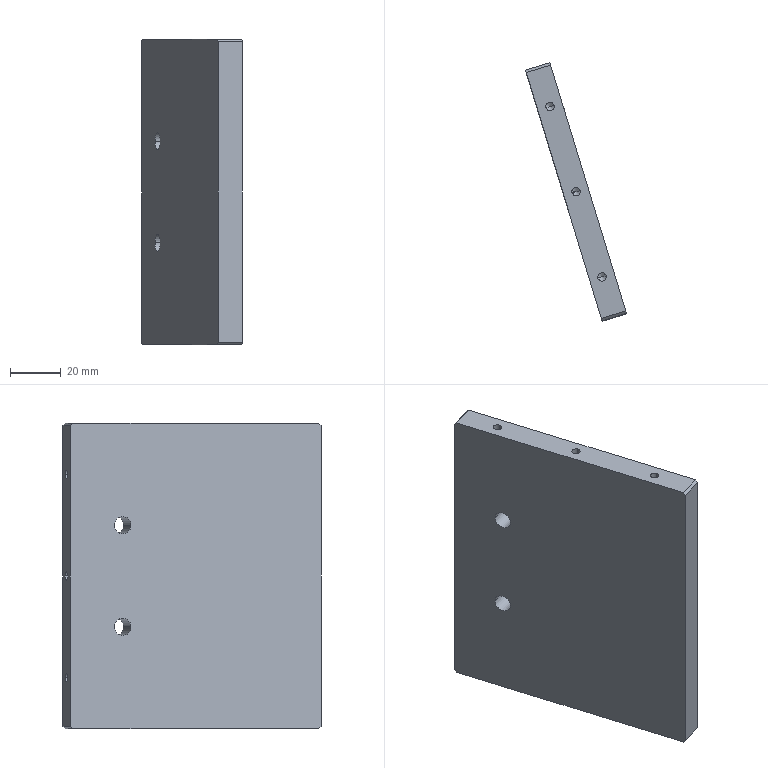Component | SolidWorks | V1ZHXTGrindingBasePlateReinforcementPlateSB1-3 | 1 solid | 38 faces | box 39.62 x 101.43 x 120 mm | volume 122318 mm3 | cylinder 16 | cone 12 | plane 10 | commonest cylinder face diameters 3.3 x12 6.8 x4
build123d program:
from build123d import *

# Parameters (mm, degrees)
SKETCH1_W             = 103
SKETCH1_H             = 120
BOSS_EXTRUDE1_DEPTH   = 5
M4_TAPPED_HOLE1_D     = 3.3
M4_TAPPED_HOLE1_DEPTH = 10.1
M4_TAPPED_HOLE1_TIP   = 0.9914
M4_TAPPED_HOLE2_D     = 3.3
M4_TAPPED_HOLE2_DEPTH = 10.1
M4_TAPPED_HOLE2_TIP   = 0.9914
M8_TAPPED_HOLE1_D     = 6.8
CHAMFER1_SIZE         = 1


with BuildPart() as part:
    # Sketch1 → Boss-Extrude1 (new, symmetric)
    with BuildSketch(Plane.XY):
        Rectangle(SKETCH1_W, SKETCH1_H)
    extrude(amount=BOSS_EXTRUDE1_DEPTH, both=True)

    # M4 Tapped Hole1
    with Locations(Plane.ZY.offset(51.5)):
        with Locations((0, 40), (0, 0), (0, -40)):
            Hole(M4_TAPPED_HOLE1_D / 2, depth=M4_TAPPED_HOLE1_DEPTH)
            with Locations((0, 0, -(M4_TAPPED_HOLE1_DEPTH + M4_TAPPED_HOLE1_TIP / 2))):  # 118° drill point
                Cone(0, M4_TAPPED_HOLE1_D / 2, M4_TAPPED_HOLE1_TIP, mode=Mode.SUBTRACT)

    # M4 Tapped Hole2
    with Locations(Plane(origin=(0, -60, 0), x_dir=(-1, 0, 0), z_dir=(0, -1, 0))):
        with Locations((35, 0), (0, 0), (-35, 0)):
            Hole(M4_TAPPED_HOLE2_D / 2, depth=M4_TAPPED_HOLE2_DEPTH)
            with Locations((0, 0, -(M4_TAPPED_HOLE2_DEPTH + M4_TAPPED_HOLE2_TIP / 2))):  # 118° drill point
                Cone(0, M4_TAPPED_HOLE2_D / 2, M4_TAPPED_HOLE2_TIP, mode=Mode.SUBTRACT)

    # M8 Tapped Hole1 (through all)
    with Locations(Plane(origin=(0, 0, -5), x_dir=(-1, 0, 0), z_dir=(0, 0, -1))):
        with Locations((30, 20), (30, -20)):
            Hole(M8_TAPPED_HOLE1_D / 2)

    # Chamfer1
    chamfer1_edges = [part.edges().sort_by_distance(p)[0] for p in [
        (51.5, -60, 0),
        (-51.5, -60, 0),
        (-51.5, 60, 0),
        (51.5, 60, 0),
    ]]
    chamfer(chamfer1_edges, length=CHAMFER1_SIZE)


solid = part.part

# Placed as in the assembly
solid = solid.moved(Location((115.024, -233.873, 375.239), (-90, 73.032, 0)))
STEP:
#1=COLOUR_RGB('',0.7922,0.8196,0.9333);
#2=FILL_AREA_STYLE_COLOUR('',#1);
#3=FILL_AREA_STYLE('',(#2));
#4=SURFACE_STYLE_FILL_AREA(#3);
#5=SURFACE_SIDE_STYLE('',(#4));
#6=SURFACE_STYLE_USAGE(.BOTH.,#5);
#7=PRESENTATION_STYLE_ASSIGNMENT((#6));
#8=CARTESIAN_POINT('',(4.411,-8.149,13.986));
#9=VERTEX_POINT('',#8);
#10=CARTESIAN_POINT('',(4.333,-7.892,13.986));
#11=VERTEX_POINT('',#10);
#12=CARTESIAN_POINT('',(4.372,-8.02,13.986));
#13=DIRECTION('',(-0.9565,-0.2918,-0.));
#14=DIRECTION('',(-0.2918,0.9565,0.));
#15=AXIS2_PLACEMENT_3D('',#12,#13,#14);
#16=CIRCLE('',#15,0.1339);
#17=EDGE_CURVE('',#9,#11,#16,.T.);
#18=ORIENTED_EDGE('',*,*,#17,.F.);
#19=CARTESIAN_POINT('',(4.035,-8.263,13.986));
#20=VERTEX_POINT('',#19);
#21=CARTESIAN_POINT('',(4.035,-8.263,13.986));
#22=DIRECTION('',(-0.9565,-0.2918,-0.));
#23=VECTOR('',#22,39.37);
#24=LINE('',#21,#23);
#25=EDGE_CURVE('',#9,#20,#24,.T.);
#26=ORIENTED_EDGE('',*,*,#25,.T.);
#27=CARTESIAN_POINT('',(3.956,-8.007,13.986));
#28=VERTEX_POINT('',#27);
#29=CARTESIAN_POINT('',(3.996,-8.135,13.986));
#30=DIRECTION('',(-0.9565,-0.2918,-0.));
#31=DIRECTION('',(-0.2918,0.9565,0.));
#32=AXIS2_PLACEMENT_3D('',#29,#30,#31);
#33=CIRCLE('',#32,0.1339);
#34=EDGE_CURVE('',#20,#28,#33,.T.);
#35=ORIENTED_EDGE('',*,*,#34,.T.);
#36=CARTESIAN_POINT('',(3.956,-8.007,13.986));
#37=DIRECTION('',(-0.9565,-0.2918,-0.));
#38=VECTOR('',#37,39.37);
#39=LINE('',#36,#38);
#40=EDGE_CURVE('',#11,#28,#39,.T.);
#41=ORIENTED_EDGE('',*,*,#40,.F.);
#42=EDGE_LOOP('',(#18,#26,#35,#41));
#43=FACE_OUTER_BOUND('',#42,.T.);
#44=CARTESIAN_POINT('',(3.996,-8.135,13.986));
#45=DIRECTION('',(-0.9565,-0.2918,-0.));
#46=DIRECTION('',(-0.2918,0.9565,0.));
#47=AXIS2_PLACEMENT_3D('',#44,#45,#46);
#48=CYLINDRICAL_SURFACE('',#47,0.1339);
#49=ADVANCED_FACE('',(#43),#48,.F.);
#50=CARTESIAN_POINT('',(4.411,-8.149,15.561));
#51=VERTEX_POINT('',#50);
#52=CARTESIAN_POINT('',(4.333,-7.892,15.561));
#53=VERTEX_POINT('',#52);
#54=CARTESIAN_POINT('',(4.372,-8.02,15.561));
#55=DIRECTION('',(-0.9565,-0.2918,-0.));
#56=DIRECTION('',(-0.2918,0.9565,0.));
#57=AXIS2_PLACEMENT_3D('',#54,#55,#56);
#58=CIRCLE('',#57,0.1339);
#59=EDGE_CURVE('',#51,#53,#58,.T.);
#60=ORIENTED_EDGE('',*,*,#59,.F.);
#61=CARTESIAN_POINT('',(4.035,-8.263,15.561));
#62=VERTEX_POINT('',#61);
#63=CARTESIAN_POINT('',(4.035,-8.263,15.561));
#64=DIRECTION('',(-0.9565,-0.2918,-0.));
#65=VECTOR('',#64,39.37);
#66=LINE('',#63,#65);
#67=EDGE_CURVE('',#51,#62,#66,.T.);
#68=ORIENTED_EDGE('',*,*,#67,.T.);
#69=CARTESIAN_POINT('',(3.956,-8.007,15.561));
#70=VERTEX_POINT('',#69);
#71=CARTESIAN_POINT('',(3.996,-8.135,15.561));
#72=DIRECTION('',(-0.9565,-0.2918,-0.));
#73=DIRECTION('',(-0.2918,0.9565,0.));
#74=AXIS2_PLACEMENT_3D('',#71,#72,#73);
#75=CIRCLE('',#74,0.1339);
#76=EDGE_CURVE('',#62,#70,#75,.T.);
#77=ORIENTED_EDGE('',*,*,#76,.T.);
#78=CARTESIAN_POINT('',(3.956,-8.007,15.561));
#79=DIRECTION('',(-0.9565,-0.2918,-0.));
#80=VECTOR('',#79,39.37);
#81=LINE('',#78,#80);
#82=EDGE_CURVE('',#53,#70,#81,.T.);
#83=ORIENTED_EDGE('',*,*,#82,.F.);
#84=EDGE_LOOP('',(#60,#68,#77,#83));
#85=FACE_OUTER_BOUND('',#84,.T.);
#86=CARTESIAN_POINT('',(3.996,-8.135,15.561));
#87=DIRECTION('',(-0.9565,-0.2918,-0.));
#88=DIRECTION('',(-0.2918,0.9565,0.));
#89=AXIS2_PLACEMENT_3D('',#86,#87,#88);
#90=CYLINDRICAL_SURFACE('',#89,0.1339);
#91=ADVANCED_FACE('',(#85),#90,.F.);
#92=CARTESIAN_POINT('',(4.188,-7.871,16.738));
#93=VERTEX_POINT('',#92);
#94=CARTESIAN_POINT('',(4.064,-7.909,16.738));
#95=VERTEX_POINT('',#94);
#96=CARTESIAN_POINT('',(4.126,-7.89,16.738));
#97=DIRECTION('',(-0.,-0.,1.));
#98=DIRECTION('',(-0.9565,-0.2918,-0.));
#99=AXIS2_PLACEMENT_3D('',#96,#97,#98);
#100=CIRCLE('',#99,0.06496);
#101=EDGE_CURVE('',#93,#95,#100,.T.);
#102=ORIENTED_EDGE('',*,*,#101,.F.);
#103=CARTESIAN_POINT('',(4.188,-7.871,17.135));
#104=VERTEX_POINT('',#103);
#105=CARTESIAN_POINT('',(4.188,-7.871,17.135));
#106=DIRECTION('',(-0.,-0.,1.));
#107=VECTOR('',#106,39.37);
#108=LINE('',#105,#107);
#109=EDGE_CURVE('',#93,#104,#108,.T.);
#110=ORIENTED_EDGE('',*,*,#109,.T.);
#111=CARTESIAN_POINT('',(4.064,-7.909,17.135));
#112=VERTEX_POINT('',#111);
#113=CARTESIAN_POINT('',(4.126,-7.89,17.135));
#114=DIRECTION('',(-0.,-0.,1.));
#115=DIRECTION('',(-0.9565,-0.2918,-0.));
#116=AXIS2_PLACEMENT_3D('',#113,#114,#115);
#117=CIRCLE('',#116,0.06496);
#118=EDGE_CURVE('',#104,#112,#117,.T.);
#119=ORIENTED_EDGE('',*,*,#118,.T.);
#120=CARTESIAN_POINT('',(4.064,-7.909,17.135));
#121=DIRECTION('',(-0.,-0.,1.));
#122=VECTOR('',#121,39.37);
#123=LINE('',#120,#122);
#124=EDGE_CURVE('',#95,#112,#123,.T.);
#125=ORIENTED_EDGE('',*,*,#124,.F.);
#126=EDGE_LOOP('',(#102,#110,#119,#125));
#127=FACE_OUTER_BOUND('',#126,.T.);
#128=CARTESIAN_POINT('',(4.126,-7.89,17.135));
#129=DIRECTION('',(-0.,-0.,1.));
#130=DIRECTION('',(-0.9565,-0.2918,-0.));
#131=AXIS2_PLACEMENT_3D('',#128,#129,#130);
#132=CYLINDRICAL_SURFACE('',#131,0.06496);
#133=ADVANCED_FACE('',(#127),#132,.F.);
#134=CARTESIAN_POINT('',(4.126,-7.89,16.699));
#135=VERTEX_POINT('',#134);
#136=CARTESIAN_POINT('',(4.064,-7.909,16.738));
#137=DIRECTION('',(-0.8199,-0.2501,0.515));
#138=VECTOR('',#137,39.37);
#139=LINE('',#136,#138);
#140=EDGE_CURVE('',#135,#95,#139,.T.);
#141=ORIENTED_EDGE('',*,*,#140,.F.);
#142=CARTESIAN_POINT('',(4.188,-7.871,16.738));
#143=DIRECTION('',(0.8199,0.2501,0.515));
#144=VECTOR('',#143,39.37);
#145=LINE('',#142,#144);
#146=EDGE_CURVE('',#135,#93,#145,.T.);
#147=ORIENTED_EDGE('',*,*,#146,.T.);
#148=ORIENTED_EDGE('',*,*,#101,.T.);
#149=EDGE_LOOP('',(#141,#147,#148));
#150=FACE_OUTER_BOUND('',#149,.T.);
#151=CARTESIAN_POINT('',(4.126,-7.89,16.738));
#152=DIRECTION('',(-0.,-0.,1.));
#153=DIRECTION('',(-0.9565,-0.2918,-0.));
#154=AXIS2_PLACEMENT_3D('',#151,#152,#153);
#155=CONICAL_SURFACE('',#154,0.06496,1.03);
#156=ADVANCED_FACE('',(#150),#155,.F.);
#157=CARTESIAN_POINT('',(4.591,-9.189,16.738));
#158=VERTEX_POINT('',#157);
#159=CARTESIAN_POINT('',(4.466,-9.227,16.738));
#160=VERTEX_POINT('',#159);
#161=CARTESIAN_POINT('',(4.528,-9.208,16.738));
#162=DIRECTION('',(-0.,-0.,1.));
#163=DIRECTION('',(-0.9565,-0.2918,-0.));
#164=AXIS2_PLACEMENT_3D('',#161,#162,#163);
#165=CIRCLE('',#164,0.06496);
#166=EDGE_CURVE('',#158,#160,#165,.T.);
#167=ORIENTED_EDGE('',*,*,#166,.F.);
#168=CARTESIAN_POINT('',(4.591,-9.189,17.135));
#169=VERTEX_POINT('',#168);
#170=CARTESIAN_POINT('',(4.591,-9.189,17.135));
#171=DIRECTION('',(-0.,-0.,1.));
#172=VECTOR('',#171,39.37);
#173=LINE('',#170,#172);
#174=EDGE_CURVE('',#158,#169,#173,.T.);
#175=ORIENTED_EDGE('',*,*,#174,.T.);
#176=CARTESIAN_POINT('',(4.466,-9.227,17.135));
#177=VERTEX_POINT('',#176);
#178=CARTESIAN_POINT('',(4.528,-9.208,17.135));
#179=DIRECTION('',(-0.,-0.,1.));
#180=DIRECTION('',(-0.9565,-0.2918,-0.));
#181=AXIS2_PLACEMENT_3D('',#178,#179,#180);
#182=CIRCLE('',#181,0.06496);
#183=EDGE_CURVE('',#169,#177,#182,.T.);
#184=ORIENTED_EDGE('',*,*,#183,.T.);
#185=CARTESIAN_POINT('',(4.466,-9.227,17.135));
#186=DIRECTION('',(-0.,-0.,1.));
#187=VECTOR('',#186,39.37);
#188=LINE('',#185,#187);
#189=EDGE_CURVE('',#160,#177,#188,.T.);
#190=ORIENTED_EDGE('',*,*,#189,.F.);
#191=EDGE_LOOP('',(#167,#175,#184,#190));
#192=FACE_OUTER_BOUND('',#191,.T.);
#193=CARTESIAN_POINT('',(4.528,-9.208,17.135));
#194=DIRECTION('',(-0.,-0.,1.));
#195=DIRECTION('',(-0.9565,-0.2918,-0.));
#196=AXIS2_PLACEMENT_3D('',#193,#194,#195);
#197=CYLINDRICAL_SURFACE('',#196,0.06496);
#198=ADVANCED_FACE('',(#192),#197,.F.);
#199=CARTESIAN_POINT('',(4.528,-9.208,16.699));
#200=VERTEX_POINT('',#199);
#201=CARTESIAN_POINT('',(4.466,-9.227,16.738));
#202=DIRECTION('',(-0.8199,-0.2501,0.515));
#203=VECTOR('',#202,39.37);
#204=LINE('',#201,#203);
#205=EDGE_CURVE('',#200,#160,#204,.T.);
#206=ORIENTED_EDGE('',*,*,#205,.F.);
#207=CARTESIAN_POINT('',(4.591,-9.189,16.738));
#208=DIRECTION('',(0.8199,0.2501,0.515));
#209=VECTOR('',#208,39.37);
#210=LINE('',#207,#209);
#211=EDGE_CURVE('',#200,#158,#210,.T.);
#212=ORIENTED_EDGE('',*,*,#211,.T.);
#213=ORIENTED_EDGE('',*,*,#166,.T.);
#214=EDGE_LOOP('',(#206,#212,#213));
#215=FACE_OUTER_BOUND('',#214,.T.);
#216=CARTESIAN_POINT('',(4.528,-9.208,16.738));
#217=DIRECTION('',(-0.,-0.,1.));
#218=DIRECTION('',(-0.9565,-0.2918,-0.));
#219=AXIS2_PLACEMENT_3D('',#216,#217,#218);
#220=CONICAL_SURFACE('',#219,0.06496,1.03);
#221=ADVANCED_FACE('',(#215),#220,.F.);
#222=CARTESIAN_POINT('',(4.993,-10.507,16.738));
#223=VERTEX_POINT('',#222);
#224=CARTESIAN_POINT('',(4.868,-10.545,16.738));
#225=VERTEX_POINT('',#224);
#226=CARTESIAN_POINT('',(4.931,-10.526,16.738));
#227=DIRECTION('',(-0.,-0.,1.));
#228=DIRECTION('',(-0.9565,-0.2918,-0.));
#229=AXIS2_PLACEMENT_3D('',#226,#227,#228);
#230=CIRCLE('',#229,0.06496);
#231=EDGE_CURVE('',#223,#225,#230,.T.);
#232=ORIENTED_EDGE('',*,*,#231,.F.);
#233=CARTESIAN_POINT('',(4.993,-10.507,17.135));
#234=VERTEX_POINT('',#233);
#235=CARTESIAN_POINT('',(4.993,-10.507,17.135));
#236=DIRECTION('',(-0.,-0.,1.));
#237=VECTOR('',#236,39.37);
#238=LINE('',#235,#237);
#239=EDGE_CURVE('',#223,#234,#238,.T.);
#240=ORIENTED_EDGE('',*,*,#239,.T.);
#241=CARTESIAN_POINT('',(4.868,-10.545,17.135));
#242=VERTEX_POINT('',#241);
#243=CARTESIAN_POINT('',(4.931,-10.526,17.135));
#244=DIRECTION('',(-0.,-0.,1.));
#245=DIRECTION('',(-0.9565,-0.2918,-0.));
#246=AXIS2_PLACEMENT_3D('',#243,#244,#245);
#247=CIRCLE('',#246,0.06496);
#248=EDGE_CURVE('',#234,#242,#247,.T.);
#249=ORIENTED_EDGE('',*,*,#248,.T.);
#250=CARTESIAN_POINT('',(4.868,-10.545,17.135));
#251=DIRECTION('',(-0.,-0.,1.));
#252=VECTOR('',#251,39.37);
#253=LINE('',#250,#252);
#254=EDGE_CURVE('',#225,#242,#253,.T.);
#255=ORIENTED_EDGE('',*,*,#254,.F.);
#256=EDGE_LOOP('',(#232,#240,#249,#255));
#257=FACE_OUTER_BOUND('',#256,.T.);
#258=CARTESIAN_POINT('',(4.931,-10.526,17.135));
#259=DIRECTION('',(-0.,-0.,1.));
#260=DIRECTION('',(-0.9565,-0.2918,-0.));
#261=AXIS2_PLACEMENT_3D('',#258,#259,#260);
#262=CYLINDRICAL_SURFACE('',#261,0.06496);
#263=ADVANCED_FACE('',(#257),#262,.F.);
#264=CARTESIAN_POINT('',(4.931,-10.526,16.699));
#265=VERTEX_POINT('',#264);
#266=CARTESIAN_POINT('',(4.868,-10.545,16.738));
#267=DIRECTION('',(-0.8199,-0.2501,0.515));
#268=VECTOR('',#267,39.37);
#269=LINE('',#266,#268);
#270=EDGE_CURVE('',#265,#225,#269,.T.);
#271=ORIENTED_EDGE('',*,*,#270,.F.);
#272=CARTESIAN_POINT('',(4.993,-10.507,16.738));
#273=DIRECTION('',(0.8199,0.2501,0.515));
#274=VECTOR('',#273,39.37);
#275=LINE('',#272,#274);
#276=EDGE_CURVE('',#265,#223,#275,.T.);
#277=ORIENTED_EDGE('',*,*,#276,.T.);
#278=ORIENTED_EDGE('',*,*,#231,.T.);
#279=EDGE_LOOP('',(#271,#277,#278));
#280=FACE_OUTER_BOUND('',#279,.T.);
#281=CARTESIAN_POINT('',(4.931,-10.526,16.738));
#282=DIRECTION('',(-0.,-0.,1.));
#283=DIRECTION('',(-0.9565,-0.2918,-0.));
#284=AXIS2_PLACEMENT_3D('',#281,#282,#283);
#285=CONICAL_SURFACE('',#284,0.06496,1.03);
#286=ADVANCED_FACE('',(#280),#285,.F.);
#287=CARTESIAN_POINT('',(3.991,-7.668,13.198));
#288=VERTEX_POINT('',#287);
#289=CARTESIAN_POINT('',(4.115,-7.63,13.198));
#290=VERTEX_POINT('',#289);
#291=CARTESIAN_POINT('',(4.053,-7.649,13.198));
#292=DIRECTION('',(-0.2918,0.9565,0.));
#293=DIRECTION('',(0.9565,0.2918,0.));
#294=AXIS2_PLACEMENT_3D('',#291,#292,#293);
#295=CIRCLE('',#294,0.06496);
#296=EDGE_CURVE('',#288,#290,#295,.T.);
#297=ORIENTED_EDGE('',*,*,#296,.F.);
#298=CARTESIAN_POINT('',(3.875,-7.287,13.198));
#299=VERTEX_POINT('',#298);
#300=CARTESIAN_POINT('',(3.875,-7.287,13.198));
#301=DIRECTION('',(-0.2918,0.9565,0.));
#302=VECTOR('',#301,39.37);
#303=LINE('',#300,#302);
#304=EDGE_CURVE('',#288,#299,#303,.T.);
#305=ORIENTED_EDGE('',*,*,#304,.T.);
#306=CARTESIAN_POINT('',(3.999,-7.249,13.198));
#307=VERTEX_POINT('',#306);
#308=CARTESIAN_POINT('',(3.937,-7.268,13.198));
#309=DIRECTION('',(-0.2918,0.9565,0.));
#310=DIRECTION('',(0.9565,0.2918,0.));
#311=AXIS2_PLACEMENT_3D('',#308,#309,#310);
#312=CIRCLE('',#311,0.06496);
#313=EDGE_CURVE('',#299,#307,#312,.T.);
#314=ORIENTED_EDGE('',*,*,#313,.T.);
#315=CARTESIAN_POINT('',(3.999,-7.249,13.198));
#316=DIRECTION('',(-0.2918,0.9565,0.));
#317=VECTOR('',#316,39.37);
#318=LINE('',#315,#317);
#319=EDGE_CURVE('',#290,#307,#318,.T.);
#320=ORIENTED_EDGE('',*,*,#319,.F.);
#321=EDGE_LOOP('',(#297,#305,#314,#320));
#322=FACE_OUTER_BOUND('',#321,.T.);
#323=CARTESIAN_POINT('',(3.937,-7.268,13.198));
#324=DIRECTION('',(-0.2918,0.9565,0.));
#325=DIRECTION('',(0.9565,0.2918,0.));
#326=AXIS2_PLACEMENT_3D('',#323,#324,#325);
#327=CYLINDRICAL_SURFACE('',#326,0.06496);
#328=ADVANCED_FACE('',(#322),#327,.F.);
#329=CARTESIAN_POINT('',(4.064,-7.686,13.198));
#330=VERTEX_POINT('',#329);
#331=CARTESIAN_POINT('',(4.115,-7.63,13.198));
#332=DIRECTION('',(0.6696,0.7428,0.));
#333=VECTOR('',#332,39.37);
#334=LINE('',#331,#333);
#335=EDGE_CURVE('',#330,#290,#334,.T.);
#336=ORIENTED_EDGE('',*,*,#335,.F.);
#337=CARTESIAN_POINT('',(3.991,-7.668,13.198));
#338=DIRECTION('',(-0.9702,0.2425,0.));
#339=VECTOR('',#338,39.37);
#340=LINE('',#337,#339);
#341=EDGE_CURVE('',#330,#288,#340,.T.);
#342=ORIENTED_EDGE('',*,*,#341,.T.);
#343=ORIENTED_EDGE('',*,*,#296,.T.);
#344=EDGE_LOOP('',(#336,#342,#343));
#345=FACE_OUTER_BOUND('',#344,.T.);
#346=CARTESIAN_POINT('',(4.053,-7.649,13.198));
#347=DIRECTION('',(-0.2918,0.9565,0.));
#348=DIRECTION('',(0.9565,0.2918,0.));
#349=AXIS2_PLACEMENT_3D('',#346,#347,#348);
#350=CONICAL_SURFACE('',#349,0.06496,1.03);
#351=ADVANCED_FACE('',(#345),#350,.F.);
#352=CARTESIAN_POINT('',(3.991,-7.668,14.773));
#353=VERTEX_POINT('',#352);
#354=CARTESIAN_POINT('',(4.115,-7.63,14.773));
#355=VERTEX_POINT('',#354);
#356=CARTESIAN_POINT('',(4.053,-7.649,14.773));
#357=DIRECTION('',(-0.2918,0.9565,0.));
#358=DIRECTION('',(0.9565,0.2918,0.));
#359=AXIS2_PLACEMENT_3D('',#356,#357,#358);
#360=CIRCLE('',#359,0.06496);
#361=EDGE_CURVE('',#353,#355,#360,.T.);
#362=ORIENTED_EDGE('',*,*,#361,.F.);
#363=CARTESIAN_POINT('',(3.875,-7.287,14.773));
#364=VERTEX_POINT('',#363);
#365=CARTESIAN_POINT('',(3.875,-7.287,14.773));
#366=DIRECTION('',(-0.2918,0.9565,0.));
#367=VECTOR('',#366,39.37);
#368=LINE('',#365,#367);
#369=EDGE_CURVE('',#353,#364,#368,.T.);
#370=ORIENTED_EDGE('',*,*,#369,.T.);
#371=CARTESIAN_POINT('',(3.999,-7.249,14.773));
#372=VERTEX_POINT('',#371);
#373=CARTESIAN_POINT('',(3.937,-7.268,14.773));
#374=DIRECTION('',(-0.2918,0.9565,0.));
#375=DIRECTION('',(0.9565,0.2918,0.));
#376=AXIS2_PLACEMENT_3D('',#373,#374,#375);
#377=CIRCLE('',#376,0.06496);
#378=EDGE_CURVE('',#364,#372,#377,.T.);
#379=ORIENTED_EDGE('',*,*,#378,.T.);
#380=CARTESIAN_POINT('',(3.999,-7.249,14.773));
#381=DIRECTION('',(-0.2918,0.9565,0.));
#382=VECTOR('',#381,39.37);
#383=LINE('',#380,#382);
#384=EDGE_CURVE('',#355,#372,#383,.T.);
#385=ORIENTED_EDGE('',*,*,#384,.F.);
#386=EDGE_LOOP('',(#362,#370,#379,#385));
#387=FACE_OUTER_BOUND('',#386,.T.);
#388=CARTESIAN_POINT('',(3.937,-7.268,14.773));
#389=DIRECTION('',(-0.2918,0.9565,0.));
#390=DIRECTION('',(0.9565,0.2918,0.));
#391=AXIS2_PLACEMENT_3D('',#388,#389,#390);
#392=CYLINDRICAL_SURFACE('',#391,0.06496);
#393=ADVANCED_FACE('',(#387),#392,.F.);
#394=CARTESIAN_POINT('',(4.064,-7.686,14.773));
#395=VERTEX_POINT('',#394);
#396=CARTESIAN_POINT('',(4.115,-7.63,14.773));
#397=DIRECTION('',(0.6696,0.7428,0.));
#398=VECTOR('',#397,39.37);
#399=LINE('',#396,#398);
#400=EDGE_CURVE('',#395,#355,#399,.T.);
#401=ORIENTED_EDGE('',*,*,#400,.F.);
#402=CARTESIAN_POINT('',(3.991,-7.668,14.773));
#403=DIRECTION('',(-0.9702,0.2425,0.));
#404=VECTOR('',#403,39.37);
#405=LINE('',#402,#404);
#406=EDGE_CURVE('',#395,#353,#405,.T.);
#407=ORIENTED_EDGE('',*,*,#406,.T.);
#408=ORIENTED_EDGE('',*,*,#361,.T.);
#409=EDGE_LOOP('',(#401,#407,#408));
#410=FACE_OUTER_BOUND('',#409,.T.);
#411=CARTESIAN_POINT('',(4.053,-7.649,14.773));
#412=DIRECTION('',(-0.2918,0.9565,0.));
#413=DIRECTION('',(0.9565,0.2918,0.));
#414=AXIS2_PLACEMENT_3D('',#411,#412,#413);
#415=CONICAL_SURFACE('',#414,0.06496,1.03);
#416=ADVANCED_FACE('',(#410),#415,.F.);
#417=CARTESIAN_POINT('',(3.991,-7.668,16.348));
#418=VERTEX_POINT('',#417);
#419=CARTESIAN_POINT('',(4.115,-7.63,16.348));
#420=VERTEX_POINT('',#419);
#421=CARTESIAN_POINT('',(4.053,-7.649,16.348));
#422=DIRECTION('',(-0.2918,0.9565,0.));
#423=DIRECTION('',(0.9565,0.2918,0.));
#424=AXIS2_PLACEMENT_3D('',#421,#422,#423);
#425=CIRCLE('',#424,0.06496);
#426=EDGE_CURVE('',#418,#420,#425,.T.);
#427=ORIENTED_EDGE('',*,*,#426,.F.);
#428=CARTESIAN_POINT('',(3.875,-7.287,16.348));
#429=VERTEX_POINT('',#428);
#430=CARTESIAN_POINT('',(3.875,-7.287,16.348));
#431=DIRECTION('',(-0.2918,0.9565,0.));
#432=VECTOR('',#431,39.37);
#433=LINE('',#430,#432);
#434=EDGE_CURVE('',#418,#429,#433,.T.);
#435=ORIENTED_EDGE('',*,*,#434,.T.);
#436=CARTESIAN_POINT('',(3.999,-7.249,16.348));
#437=VERTEX_POINT('',#436);
#438=CARTESIAN_POINT('',(3.937,-7.268,16.348));
#439=DIRECTION('',(-0.2918,0.9565,0.));
#440=DIRECTION('',(0.9565,0.2918,0.));
#441=AXIS2_PLACEMENT_3D('',#438,#439,#440);
#442=CIRCLE('',#441,0.06496);
#443=EDGE_CURVE('',#429,#437,#442,.T.);
#444=ORIENTED_EDGE('',*,*,#443,.T.);
#445=CARTESIAN_POINT('',(3.999,-7.249,16.348));
#446=DIRECTION('',(-0.2918,0.9565,0.));
#447=VECTOR('',#446,39.37);
#448=LINE('',#445,#447);
#449=EDGE_CURVE('',#420,#437,#448,.T.);
#450=ORIENTED_EDGE('',*,*,#449,.F.);
#451=EDGE_LOOP('',(#427,#435,#444,#450));
#452=FACE_OUTER_BOUND('',#451,.T.);
#453=CARTESIAN_POINT('',(3.937,-7.268,16.348));
#454=DIRECTION('',(-0.2918,0.9565,0.));
#455=DIRECTION('',(0.9565,0.2918,0.));
#456=AXIS2_PLACEMENT_3D('',#453,#454,#455);
#457=CYLINDRICAL_SURFACE('',#456,0.06496);
#458=ADVANCED_FACE('',(#452),#457,.F.);
#459=CARTESIAN_POINT('',(4.064,-7.686,16.348));
#460=VERTEX_POINT('',#459);
#461=CARTESIAN_POINT('',(4.115,-7.63,16.348));
#462=DIRECTION('',(0.6696,0.7428,0.));
#463=VECTOR('',#462,39.37);
#464=LINE('',#461,#463);
#465=EDGE_CURVE('',#460,#420,#464,.T.);
#466=ORIENTED_EDGE('',*,*,#465,.F.);
#467=CARTESIAN_POINT('',(3.991,-7.668,16.348));
#468=DIRECTION('',(-0.9702,0.2425,0.));
#469=VECTOR('',#468,39.37);
#470=LINE('',#467,#469);
#471=EDGE_CURVE('',#460,#418,#470,.T.);
#472=ORIENTED_EDGE('',*,*,#471,.T.);
#473=ORIENTED_EDGE('',*,*,#426,.T.);
#474=EDGE_LOOP('',(#466,#472,#473));
#475=FACE_OUTER_BOUND('',#474,.T.);
#476=CARTESIAN_POINT('',(4.053,-7.649,16.348));
#477=DIRECTION('',(-0.2918,0.9565,0.));
#478=DIRECTION('',(0.9565,0.2918,0.));
#479=AXIS2_PLACEMENT_3D('',#476,#477,#478);
#480=CONICAL_SURFACE('',#479,0.06496,1.03);
#481=ADVANCED_FACE('',(#475),#480,.F.);
#482=CARTESIAN_POINT('',(5.308,-11.089,17.096));
#483=VERTEX_POINT('',#482);
#484=CARTESIAN_POINT('',(5.308,-11.089,12.45));
#485=VERTEX_POINT('',#484);
#486=CARTESIAN_POINT('',(5.308,-11.089,17.135));
#487=DIRECTION('',(0.,0.,-1.));
#488=VECTOR('',#487,39.37);
#489=LINE('',#486,#488);
#490=EDGE_CURVE('',#483,#485,#489,.T.);
#491=ORIENTED_EDGE('',*,*,#490,.F.);
#492=CARTESIAN_POINT('',(4.932,-11.204,17.096));
#493=VERTEX_POINT('',#492);
#494=CARTESIAN_POINT('',(5.308,-11.089,17.096));
#495=DIRECTION('',(-0.9565,-0.2918,-0.));
#496=VECTOR('',#495,39.37);
#497=LINE('',#494,#496);
#498=EDGE_CURVE('',#483,#493,#497,.T.);
#499=ORIENTED_EDGE('',*,*,#498,.T.);
#500=CARTESIAN_POINT('',(4.932,-11.204,12.45));
#501=VERTEX_POINT('',#500);
#502=CARTESIAN_POINT('',(4.932,-11.204,17.135));
#503=DIRECTION('',(0.,0.,-1.));
#504=VECTOR('',#503,39.37);
#505=LINE('',#502,#504);
#506=EDGE_CURVE('',#493,#501,#505,.T.);
#507=ORIENTED_EDGE('',*,*,#506,.T.);
#508=CARTESIAN_POINT('',(5.308,-11.089,12.45));
#509=DIRECTION('',(0.9565,0.2918,0.));
#510=VECTOR('',#509,39.37);
#511=LINE('',#508,#510);
#512=EDGE_CURVE('',#501,#485,#511,.T.);
#513=ORIENTED_EDGE('',*,*,#512,.T.);
#514=EDGE_LOOP('',(#491,#499,#507,#513));
#515=FACE_OUTER_BOUND('',#514,.T.);
#516=CARTESIAN_POINT('',(5.308,-11.089,17.135));
#517=DIRECTION('',(-0.2918,0.9565,0.));
#518=DIRECTION('',(0.9565,0.2918,0.));
#519=AXIS2_PLACEMENT_3D('',#516,#517,#518);
#520=PLANE('',#519);
#521=ADVANCED_FACE('',(#515),#520,.F.);
#522=CARTESIAN_POINT('',(5.297,-11.052,12.411));
#523=VERTEX_POINT('',#522);
#524=CARTESIAN_POINT('',(4.137,-7.249,12.411));
#525=VERTEX_POINT('',#524);
#526=CARTESIAN_POINT('',(4.125,-7.211,12.411));
#527=DIRECTION('',(-0.2918,0.9565,0.));
#528=VECTOR('',#527,39.37);
#529=LINE('',#526,#528);
#530=EDGE_CURVE('',#523,#525,#529,.T.);
#531=ORIENTED_EDGE('',*,*,#530,.F.);
#532=CARTESIAN_POINT('',(4.92,-11.167,12.411));
#533=VERTEX_POINT('',#532);
#534=CARTESIAN_POINT('',(5.297,-11.052,12.411));
#535=DIRECTION('',(-0.9565,-0.2918,-0.));
#536=VECTOR('',#535,39.37);
#537=LINE('',#534,#536);
#538=EDGE_CURVE('',#523,#533,#537,.T.);
#539=ORIENTED_EDGE('',*,*,#538,.T.);
#540=CARTESIAN_POINT('',(3.76,-7.363,12.411));
#541=VERTEX_POINT('',#540);
#542=CARTESIAN_POINT('',(3.749,-7.326,12.411));
#543=DIRECTION('',(-0.2918,0.9565,0.));
#544=VECTOR('',#543,39.37);
#545=LINE('',#542,#544);
#546=EDGE_CURVE('',#533,#541,#545,.T.);
#547=ORIENTED_EDGE('',*,*,#546,.T.);
#548=CARTESIAN_POINT('',(4.137,-7.249,12.411));
#549=DIRECTION('',(0.9565,0.2918,0.));
#550=VECTOR('',#549,39.37);
#551=LINE('',#548,#550);
#552=EDGE_CURVE('',#541,#525,#551,.T.);
#553=ORIENTED_EDGE('',*,*,#552,.T.);
#554=EDGE_LOOP('',(#531,#539,#547,#553));
#555=FACE_OUTER_BOUND('',#554,.T.);
#556=CARTESIAN_POINT('',(4.125,-7.211,12.411));
#557=DIRECTION('',(-0.,-0.,1.));
#558=DIRECTION('',(-0.9565,-0.2918,-0.));
#559=AXIS2_PLACEMENT_3D('',#556,#557,#558);
#560=PLANE('',#559);
#561=ADVANCED_FACE('',(#555),#560,.F.);
#562=CARTESIAN_POINT('',(3.937,-7.268,13.198));
#563=DIRECTION('',(-0.2918,0.9565,0.));
#564=DIRECTION('',(0.9565,0.2918,0.));
#565=AXIS2_PLACEMENT_3D('',#562,#563,#564);
#566=CIRCLE('',#565,0.06496);
#567=EDGE_CURVE('',#307,#299,#566,.T.);
#568=ORIENTED_EDGE('',*,*,#567,.F.);
#569=ORIENTED_EDGE('',*,*,#313,.F.);
#570=EDGE_LOOP('',(#568,#569));
#571=FACE_BOUND('',#570,.T.);
#572=CARTESIAN_POINT('',(3.937,-7.268,14.773));
#573=DIRECTION('',(-0.2918,0.9565,0.));
#574=DIRECTION('',(0.9565,0.2918,0.));
#575=AXIS2_PLACEMENT_3D('',#572,#573,#574);
#576=CIRCLE('',#575,0.06496);
#577=EDGE_CURVE('',#372,#364,#576,.T.);
#578=ORIENTED_EDGE('',*,*,#577,.F.);
#579=ORIENTED_EDGE('',*,*,#378,.F.);
#580=EDGE_LOOP('',(#578,#579));
#581=FACE_BOUND('',#580,.T.);
#582=CARTESIAN_POINT('',(3.937,-7.268,16.348));
#583=DIRECTION('',(-0.2918,0.9565,0.));
#584=DIRECTION('',(0.9565,0.2918,0.));
#585=AXIS2_PLACEMENT_3D('',#582,#583,#584);
#586=CIRCLE('',#585,0.06496);
#587=EDGE_CURVE('',#437,#429,#586,.T.);
#588=ORIENTED_EDGE('',*,*,#587,.F.);
#589=ORIENTED_EDGE('',*,*,#443,.F.);
#590=EDGE_LOOP('',(#588,#589));
#591=FACE_BOUND('',#590,.T.);
#592=CARTESIAN_POINT('',(3.749,-7.326,12.45));
#593=VERTEX_POINT('',#592);
#594=CARTESIAN_POINT('',(3.749,-7.326,17.096));
#595=VERTEX_POINT('',#594);
#596=CARTESIAN_POINT('',(3.749,-7.326,17.135));
#597=DIRECTION('',(-0.,-0.,1.));
#598=VECTOR('',#597,39.37);
#599=LINE('',#596,#598);
#600=EDGE_CURVE('',#593,#595,#599,.T.);
#601=ORIENTED_EDGE('',*,*,#600,.T.);
#602=CARTESIAN_POINT('',(4.125,-7.211,17.096));
#603=VERTEX_POINT('',#602);
#604=CARTESIAN_POINT('',(4.125,-7.211,17.096));
#605=DIRECTION('',(0.9565,0.2918,0.));
#606=VECTOR('',#605,39.37);
#607=LINE('',#604,#606);
#608=EDGE_CURVE('',#595,#603,#607,.T.);
#609=ORIENTED_EDGE('',*,*,#608,.T.);
#610=CARTESIAN_POINT('',(4.125,-7.211,12.45));
#611=VERTEX_POINT('',#610);
#612=CARTESIAN_POINT('',(4.125,-7.211,17.135));
#613=DIRECTION('',(-0.,-0.,1.));
#614=VECTOR('',#613,39.37);
#615=LINE('',#612,#614);
#616=EDGE_CURVE('',#611,#603,#615,.T.);
#617=ORIENTED_EDGE('',*,*,#616,.F.);
#618=CARTESIAN_POINT('',(4.125,-7.211,12.45));
#619=DIRECTION('',(-0.9565,-0.2918,-0.));
#620=VECTOR('',#619,39.37);
#621=LINE('',#618,#620);
#622=EDGE_CURVE('',#611,#593,#621,.T.);
#623=ORIENTED_EDGE('',*,*,#622,.T.);
#624=EDGE_LOOP('',(#601,#609,#617,#623));
#625=FACE_OUTER_BOUND('',#624,.T.);
#626=CARTESIAN_POINT('',(4.125,-7.211,17.135));
#627=DIRECTION('',(0.2918,-0.9565,-0.));
#628=DIRECTION('',(-0.9565,-0.2918,-0.));
#629=AXIS2_PLACEMENT_3D('',#626,#627,#628);
#630=PLANE('',#629);
#631=ADVANCED_FACE('',(#571,#581,#591,#625),#630,.F.);
#632=CARTESIAN_POINT('',(4.126,-7.89,17.135));
#633=DIRECTION('',(-0.,-0.,1.));
#634=DIRECTION('',(-0.9565,-0.2918,-0.));
#635=AXIS2_PLACEMENT_3D('',#632,#633,#634);
#636=CIRCLE('',#635,0.06496);
#637=EDGE_CURVE('',#112,#104,#636,.T.);
#638=ORIENTED_EDGE('',*,*,#637,.F.);
#639=ORIENTED_EDGE('',*,*,#118,.F.);
#640=EDGE_LOOP('',(#638,#639));
#641=FACE_BOUND('',#640,.T.);
#642=CARTESIAN_POINT('',(4.528,-9.208,17.135));
#643=DIRECTION('',(-0.,-0.,1.));
#644=DIRECTION('',(-0.9565,-0.2918,-0.));
#645=AXIS2_PLACEMENT_3D('',#642,#643,#644);
#646=CIRCLE('',#645,0.06496);
#647=EDGE_CURVE('',#177,#169,#646,.T.);
#648=ORIENTED_EDGE('',*,*,#647,.F.);
#649=ORIENTED_EDGE('',*,*,#183,.F.);
#650=EDGE_LOOP('',(#648,#649));
#651=FACE_BOUND('',#650,.T.);
#652=CARTESIAN_POINT('',(4.931,-10.526,17.135));
#653=DIRECTION('',(-0.,-0.,1.));
#654=DIRECTION('',(-0.9565,-0.2918,-0.));
#655=AXIS2_PLACEMENT_3D('',#652,#653,#654);
#656=CIRCLE('',#655,0.06496);
#657=EDGE_CURVE('',#242,#234,#656,.T.);
#658=ORIENTED_EDGE('',*,*,#657,.F.);
#659=ORIENTED_EDGE('',*,*,#248,.F.);
#660=EDGE_LOOP('',(#658,#659));
#661=FACE_BOUND('',#660,.T.);
#662=CARTESIAN_POINT('',(4.137,-7.249,17.135));
#663=VERTEX_POINT('',#662);
#664=CARTESIAN_POINT('',(5.297,-11.052,17.135));
#665=VERTEX_POINT('',#664);
#666=CARTESIAN_POINT('',(4.125,-7.211,17.135));
#667=DIRECTION('',(0.2918,-0.9565,-0.));
#668=VECTOR('',#667,39.37);
#669=LINE('',#666,#668);
#670=EDGE_CURVE('',#663,#665,#669,.T.);
#671=ORIENTED_EDGE('',*,*,#670,.F.);
#672=CARTESIAN_POINT('',(3.76,-7.363,17.135));
#673=VERTEX_POINT('',#672);
#674=CARTESIAN_POINT('',(4.137,-7.249,17.135));
#675=DIRECTION('',(-0.9565,-0.2918,-0.));
#676=VECTOR('',#675,39.37);
#677=LINE('',#674,#676);
#678=EDGE_CURVE('',#663,#673,#677,.T.);
#679=ORIENTED_EDGE('',*,*,#678,.T.);
#680=CARTESIAN_POINT('',(4.92,-11.167,17.135));
#681=VERTEX_POINT('',#680);
#682=CARTESIAN_POINT('',(3.749,-7.326,17.135));
#683=DIRECTION('',(0.2918,-0.9565,-0.));
#684=VECTOR('',#683,39.37);
#685=LINE('',#682,#684);
#686=EDGE_CURVE('',#673,#681,#685,.T.);
#687=ORIENTED_EDGE('',*,*,#686,.T.);
#688=CARTESIAN_POINT('',(5.297,-11.052,17.135));
#689=DIRECTION('',(0.9565,0.2918,0.));
#690=VECTOR('',#689,39.37);
#691=LINE('',#688,#690);
#692=EDGE_CURVE('',#681,#665,#691,.T.);
#693=ORIENTED_EDGE('',*,*,#692,.T.);
#694=EDGE_LOOP('',(#671,#679,#687,#693));
#695=FACE_OUTER_BOUND('',#694,.T.);
#696=CARTESIAN_POINT('',(4.125,-7.211,17.135));
#697=DIRECTION('',(0.,0.,-1.));
#698=DIRECTION('',(0.9565,0.2918,0.));
#699=AXIS2_PLACEMENT_3D('',#696,#697,#698);
#700=PLANE('',#699);
#701=ADVANCED_FACE('',(#641,#651,#661,#695),#700,.F.);
#702=CARTESIAN_POINT('',(4.372,-8.02,13.986));
#703=DIRECTION('',(-0.9565,-0.2918,-0.));
#704=DIRECTION('',(-0.2918,0.9565,0.));
#705=AXIS2_PLACEMENT_3D('',#702,#703,#704);
#706=CIRCLE('',#705,0.1339);
#707=EDGE_CURVE('',#11,#9,#706,.T.);
#708=ORIENTED_EDGE('',*,*,#707,.T.);
#709=ORIENTED_EDGE('',*,*,#17,.T.);
#710=EDGE_LOOP('',(#708,#709));
#711=FACE_BOUND('',#710,.T.);
#712=CARTESIAN_POINT('',(4.372,-8.02,15.561));
#713=DIRECTION('',(-0.9565,-0.2918,-0.));
#714=DIRECTION('',(-0.2918,0.9565,0.));
#715=AXIS2_PLACEMENT_3D('',#712,#713,#714);
#716=CIRCLE('',#715,0.1339);
#717=EDGE_CURVE('',#53,#51,#716,.T.);
#718=ORIENTED_EDGE('',*,*,#717,.T.);
#719=ORIENTED_EDGE('',*,*,#59,.T.);
#720=EDGE_LOOP('',(#718,#719));
#721=FACE_BOUND('',#720,.T.);
#722=ORIENTED_EDGE('',*,*,#616,.T.);
#723=CARTESIAN_POINT('',(4.137,-7.249,17.135));
#724=DIRECTION('',(0.2064,-0.6763,0.7071));
#725=VECTOR('',#724,39.37);
#726=LINE('',#723,#725);
#727=EDGE_CURVE('',#603,#663,#726,.T.);
#728=ORIENTED_EDGE('',*,*,#727,.T.);
#729=ORIENTED_EDGE('',*,*,#670,.T.);
#730=CARTESIAN_POINT('',(5.308,-11.089,17.096));
#731=DIRECTION('',(0.2064,-0.6763,-0.7071));
#732=VECTOR('',#731,39.37);
#733=LINE('',#730,#732);
#734=EDGE_CURVE('',#665,#483,#733,.T.);
#735=ORIENTED_EDGE('',*,*,#734,.T.);
#736=ORIENTED_EDGE('',*,*,#490,.T.);
#737=CARTESIAN_POINT('',(5.297,-11.052,12.411));
#738=DIRECTION('',(-0.2064,0.6763,-0.7071));
#739=VECTOR('',#738,39.37);
#740=LINE('',#737,#739);
#741=EDGE_CURVE('',#485,#523,#740,.T.);
#742=ORIENTED_EDGE('',*,*,#741,.T.);
#743=ORIENTED_EDGE('',*,*,#530,.T.);
#744=CARTESIAN_POINT('',(4.125,-7.211,12.45));
#745=DIRECTION('',(-0.2064,0.6763,0.7071));
#746=VECTOR('',#745,39.37);
#747=LINE('',#744,#746);
#748=EDGE_CURVE('',#525,#611,#747,.T.);
#749=ORIENTED_EDGE('',*,*,#748,.T.);
#750=EDGE_LOOP('',(#722,#728,#729,#735,#736,#742,#743,#749));
#751=FACE_OUTER_BOUND('',#750,.T.);
#752=CARTESIAN_POINT('',(4.717,-9.15,14.773));
#753=DIRECTION('',(-0.9565,-0.2918,-0.));
#754=DIRECTION('',(-0.2918,0.9565,0.));
#755=AXIS2_PLACEMENT_3D('',#752,#753,#754);
#756=PLANE('',#755);
#757=ADVANCED_FACE('',(#711,#721,#751),#756,.F.);
#758=CARTESIAN_POINT('',(3.996,-8.135,13.986));
#759=DIRECTION('',(-0.9565,-0.2918,-0.));
#760=DIRECTION('',(-0.2918,0.9565,0.));
#761=AXIS2_PLACEMENT_3D('',#758,#759,#760);
#762=CIRCLE('',#761,0.1339);
#763=EDGE_CURVE('',#28,#20,#762,.T.);
#764=ORIENTED_EDGE('',*,*,#763,.F.);
#765=ORIENTED_EDGE('',*,*,#34,.F.);
#766=EDGE_LOOP('',(#764,#765));
#767=FACE_BOUND('',#766,.T.);
#768=CARTESIAN_POINT('',(3.996,-8.135,15.561));
#769=DIRECTION('',(-0.9565,-0.2918,-0.));
#770=DIRECTION('',(-0.2918,0.9565,0.));
#771=AXIS2_PLACEMENT_3D('',#768,#769,#770);
#772=CIRCLE('',#771,0.1339);
#773=EDGE_CURVE('',#70,#62,#772,.T.);
#774=ORIENTED_EDGE('',*,*,#773,.F.);
#775=ORIENTED_EDGE('',*,*,#76,.F.);
#776=EDGE_LOOP('',(#774,#775));
#777=FACE_BOUND('',#776,.T.);
#778=ORIENTED_EDGE('',*,*,#686,.F.);
#779=CARTESIAN_POINT('',(3.705,-7.185,16.948));
#780=DIRECTION('',(-0.2064,0.6763,-0.7071));
#781=VECTOR('',#780,39.37);
#782=LINE('',#779,#781);
#783=EDGE_CURVE('',#673,#595,#782,.T.);
#784=ORIENTED_EDGE('',*,*,#783,.T.);
#785=ORIENTED_EDGE('',*,*,#600,.F.);
#786=CARTESIAN_POINT('',(3.705,-7.185,12.598));
#787=DIRECTION('',(0.2064,-0.6763,-0.7071));
#788=VECTOR('',#787,39.37);
#789=LINE('',#786,#788);
#790=EDGE_CURVE('',#593,#541,#789,.T.);
#791=ORIENTED_EDGE('',*,*,#790,.T.);
#792=ORIENTED_EDGE('',*,*,#546,.F.);
#793=CARTESIAN_POINT('',(4.975,-11.346,12.598));
#794=DIRECTION('',(0.2064,-0.6763,0.7071));
#795=VECTOR('',#794,39.37);
#796=LINE('',#793,#795);
#797=EDGE_CURVE('',#533,#501,#796,.T.);
#798=ORIENTED_EDGE('',*,*,#797,.T.);
#799=ORIENTED_EDGE('',*,*,#506,.F.);
#800=CARTESIAN_POINT('',(4.975,-11.346,16.948));
#801=DIRECTION('',(-0.2064,0.6763,0.7071));
#802=VECTOR('',#801,39.37);
#803=LINE('',#800,#802);
#804=EDGE_CURVE('',#493,#681,#803,.T.);
#805=ORIENTED_EDGE('',*,*,#804,.T.);
#806=EDGE_LOOP('',(#778,#784,#785,#791,#792,#798,#799,#805));
#807=FACE_OUTER_BOUND('',#806,.T.);
#808=CARTESIAN_POINT('',(4.34,-9.265,14.773));
#809=DIRECTION('',(-0.9565,-0.2918,-0.));
#810=DIRECTION('',(-0.2918,0.9565,0.));
#811=AXIS2_PLACEMENT_3D('',#808,#809,#810);
#812=PLANE('',#811);
#813=ADVANCED_FACE('',(#767,#777,#807),#812,.T.);
#814=ORIENTED_EDGE('',*,*,#471,.F.);
#815=ORIENTED_EDGE('',*,*,#465,.T.);
#816=CARTESIAN_POINT('',(4.053,-7.649,16.348));
#817=DIRECTION('',(-0.2918,0.9565,0.));
#818=DIRECTION('',(0.9565,0.2918,0.));
#819=AXIS2_PLACEMENT_3D('',#816,#817,#818);
#820=CIRCLE('',#819,0.06496);
#821=EDGE_CURVE('',#420,#418,#820,.T.);
#822=ORIENTED_EDGE('',*,*,#821,.T.);
#823=EDGE_LOOP('',(#814,#815,#822));
#824=FACE_OUTER_BOUND('',#823,.T.);
#825=CARTESIAN_POINT('',(4.053,-7.649,16.348));
#826=DIRECTION('',(-0.2918,0.9565,0.));
#827=DIRECTION('',(0.9565,0.2918,0.));
#828=AXIS2_PLACEMENT_3D('',#825,#826,#827);
#829=CONICAL_SURFACE('',#828,0.06496,1.03);
#830=ADVANCED_FACE('',(#824),#829,.F.);
#831=ORIENTED_EDGE('',*,*,#434,.F.);
#832=ORIENTED_EDGE('',*,*,#821,.F.);
#833=ORIENTED_EDGE('',*,*,#449,.T.);
#834=ORIENTED_EDGE('',*,*,#587,.T.);
#835=EDGE_LOOP('',(#831,#832,#833,#834));
#836=FACE_OUTER_BOUND('',#835,.T.);
#837=CARTESIAN_POINT('',(3.937,-7.268,16.348));
#838=DIRECTION('',(-0.2918,0.9565,0.));
#839=DIRECTION('',(0.9565,0.2918,0.));
#840=AXIS2_PLACEMENT_3D('',#837,#838,#839);
#841=CYLINDRICAL_SURFACE('',#840,0.06496);
#842=ADVANCED_FACE('',(#836),#841,.F.);
#843=ORIENTED_EDGE('',*,*,#406,.F.);
#844=ORIENTED_EDGE('',*,*,#400,.T.);
#845=CARTESIAN_POINT('',(4.053,-7.649,14.773));
#846=DIRECTION('',(-0.2918,0.9565,0.));
#847=DIRECTION('',(0.9565,0.2918,0.));
#848=AXIS2_PLACEMENT_3D('',#845,#846,#847);
#849=CIRCLE('',#848,0.06496);
#850=EDGE_CURVE('',#355,#353,#849,.T.);
#851=ORIENTED_EDGE('',*,*,#850,.T.);
#852=EDGE_LOOP('',(#843,#844,#851));
#853=FACE_OUTER_BOUND('',#852,.T.);
#854=CARTESIAN_POINT('',(4.053,-7.649,14.773));
#855=DIRECTION('',(-0.2918,0.9565,0.));
#856=DIRECTION('',(0.9565,0.2918,0.));
#857=AXIS2_PLACEMENT_3D('',#854,#855,#856);
#858=CONICAL_SURFACE('',#857,0.06496,1.03);
#859=ADVANCED_FACE('',(#853),#858,.F.);
#860=ORIENTED_EDGE('',*,*,#369,.F.);
#861=ORIENTED_EDGE('',*,*,#850,.F.);
#862=ORIENTED_EDGE('',*,*,#384,.T.);
#863=ORIENTED_EDGE('',*,*,#577,.T.);
#864=EDGE_LOOP('',(#860,#861,#862,#863));
#865=FACE_OUTER_BOUND('',#864,.T.);
#866=CARTESIAN_POINT('',(3.937,-7.268,14.773));
#867=DIRECTION('',(-0.2918,0.9565,0.));
#868=DIRECTION('',(0.9565,0.2918,0.));
#869=AXIS2_PLACEMENT_3D('',#866,#867,#868);
#870=CYLINDRICAL_SURFACE('',#869,0.06496);
#871=ADVANCED_FACE('',(#865),#870,.F.);
#872=ORIENTED_EDGE('',*,*,#341,.F.);
#873=ORIENTED_EDGE('',*,*,#335,.T.);
#874=CARTESIAN_POINT('',(4.053,-7.649,13.198));
#875=DIRECTION('',(-0.2918,0.9565,0.));
#876=DIRECTION('',(0.9565,0.2918,0.));
#877=AXIS2_PLACEMENT_3D('',#874,#875,#876);
#878=CIRCLE('',#877,0.06496);
#879=EDGE_CURVE('',#290,#288,#878,.T.);
#880=ORIENTED_EDGE('',*,*,#879,.T.);
#881=EDGE_LOOP('',(#872,#873,#880));
#882=FACE_OUTER_BOUND('',#881,.T.);
#883=CARTESIAN_POINT('',(4.053,-7.649,13.198));
#884=DIRECTION('',(-0.2918,0.9565,0.));
#885=DIRECTION('',(0.9565,0.2918,0.));
#886=AXIS2_PLACEMENT_3D('',#883,#884,#885);
#887=CONICAL_SURFACE('',#886,0.06496,1.03);
#888=ADVANCED_FACE('',(#882),#887,.F.);
#889=ORIENTED_EDGE('',*,*,#304,.F.);
#890=ORIENTED_EDGE('',*,*,#879,.F.);
#891=ORIENTED_EDGE('',*,*,#319,.T.);
#892=ORIENTED_EDGE('',*,*,#567,.T.);
#893=EDGE_LOOP('',(#889,#890,#891,#892));
#894=FACE_OUTER_BOUND('',#893,.T.);
#895=CARTESIAN_POINT('',(3.937,-7.268,13.198));
#896=DIRECTION('',(-0.2918,0.9565,0.));
#897=DIRECTION('',(0.9565,0.2918,0.));
#898=AXIS2_PLACEMENT_3D('',#895,#896,#897);
#899=CYLINDRICAL_SURFACE('',#898,0.06496);
#900=ADVANCED_FACE('',(#894),#899,.F.);
#901=ORIENTED_EDGE('',*,*,#276,.F.);
#902=ORIENTED_EDGE('',*,*,#270,.T.);
#903=CARTESIAN_POINT('',(4.931,-10.526,16.738));
#904=DIRECTION('',(-0.,-0.,1.));
#905=DIRECTION('',(-0.9565,-0.2918,-0.));
#906=AXIS2_PLACEMENT_3D('',#903,#904,#905);
#907=CIRCLE('',#906,0.06496);
#908=EDGE_CURVE('',#225,#223,#907,.T.);
#909=ORIENTED_EDGE('',*,*,#908,.T.);
#910=EDGE_LOOP('',(#901,#902,#909));
#911=FACE_OUTER_BOUND('',#910,.T.);
#912=CARTESIAN_POINT('',(4.931,-10.526,16.738));
#913=DIRECTION('',(-0.,-0.,1.));
#914=DIRECTION('',(-0.9565,-0.2918,-0.));
#915=AXIS2_PLACEMENT_3D('',#912,#913,#914);
#916=CONICAL_SURFACE('',#915,0.06496,1.03);
#917=ADVANCED_FACE('',(#911),#916,.F.);
#918=ORIENTED_EDGE('',*,*,#239,.F.);
#919=ORIENTED_EDGE('',*,*,#908,.F.);
#920=ORIENTED_EDGE('',*,*,#254,.T.);
#921=ORIENTED_EDGE('',*,*,#657,.T.);
#922=EDGE_LOOP('',(#918,#919,#920,#921));
#923=FACE_OUTER_BOUND('',#922,.T.);
#924=CARTESIAN_POINT('',(4.931,-10.526,17.135));
#925=DIRECTION('',(-0.,-0.,1.));
#926=DIRECTION('',(-0.9565,-0.2918,-0.));
#927=AXIS2_PLACEMENT_3D('',#924,#925,#926);
#928=CYLINDRICAL_SURFACE('',#927,0.06496);
#929=ADVANCED_FACE('',(#923),#928,.F.);
#930=ORIENTED_EDGE('',*,*,#211,.F.);
#931=ORIENTED_EDGE('',*,*,#205,.T.);
#932=CARTESIAN_POINT('',(4.528,-9.208,16.738));
#933=DIRECTION('',(-0.,-0.,1.));
#934=DIRECTION('',(-0.9565,-0.2918,-0.));
#935=AXIS2_PLACEMENT_3D('',#932,#933,#934);
#936=CIRCLE('',#935,0.06496);
#937=EDGE_CURVE('',#160,#158,#936,.T.);
#938=ORIENTED_EDGE('',*,*,#937,.T.);
#939=EDGE_LOOP('',(#930,#931,#938));
#940=FACE_OUTER_BOUND('',#939,.T.);
#941=CARTESIAN_POINT('',(4.528,-9.208,16.738));
#942=DIRECTION('',(-0.,-0.,1.));
#943=DIRECTION('',(-0.9565,-0.2918,-0.));
#944=AXIS2_PLACEMENT_3D('',#941,#942,#943);
#945=CONICAL_SURFACE('',#944,0.06496,1.03);
#946=ADVANCED_FACE('',(#940),#945,.F.);
#947=ORIENTED_EDGE('',*,*,#174,.F.);
#948=ORIENTED_EDGE('',*,*,#937,.F.);
#949=ORIENTED_EDGE('',*,*,#189,.T.);
#950=ORIENTED_EDGE('',*,*,#647,.T.);
#951=EDGE_LOOP('',(#947,#948,#949,#950));
#952=FACE_OUTER_BOUND('',#951,.T.);
#953=CARTESIAN_POINT('',(4.528,-9.208,17.135));
#954=DIRECTION('',(-0.,-0.,1.));
#955=DIRECTION('',(-0.9565,-0.2918,-0.));
#956=AXIS2_PLACEMENT_3D('',#953,#954,#955);
#957=CYLINDRICAL_SURFACE('',#956,0.06496);
#958=ADVANCED_FACE('',(#952),#957,.F.);
#959=ORIENTED_EDGE('',*,*,#146,.F.);
#960=ORIENTED_EDGE('',*,*,#140,.T.);
#961=CARTESIAN_POINT('',(4.126,-7.89,16.738));
#962=DIRECTION('',(-0.,-0.,1.));
#963=DIRECTION('',(-0.9565,-0.2918,-0.));
#964=AXIS2_PLACEMENT_3D('',#961,#962,#963);
#965=CIRCLE('',#964,0.06496);
#966=EDGE_CURVE('',#95,#93,#965,.T.);
#967=ORIENTED_EDGE('',*,*,#966,.T.);
#968=EDGE_LOOP('',(#959,#960,#967));
#969=FACE_OUTER_BOUND('',#968,.T.);
#970=CARTESIAN_POINT('',(4.126,-7.89,16.738));
#971=DIRECTION('',(-0.,-0.,1.));
#972=DIRECTION('',(-0.9565,-0.2918,-0.));
#973=AXIS2_PLACEMENT_3D('',#970,#971,#972);
#974=CONICAL_SURFACE('',#973,0.06496,1.03);
#975=ADVANCED_FACE('',(#969),#974,.F.);
#976=ORIENTED_EDGE('',*,*,#109,.F.);
#977=ORIENTED_EDGE('',*,*,#966,.F.);
#978=ORIENTED_EDGE('',*,*,#124,.T.);
#979=ORIENTED_EDGE('',*,*,#637,.T.);
#980=EDGE_LOOP('',(#976,#977,#978,#979));
#981=FACE_OUTER_BOUND('',#980,.T.);
#982=CARTESIAN_POINT('',(4.126,-7.89,17.135));
#983=DIRECTION('',(-0.,-0.,1.));
#984=DIRECTION('',(-0.9565,-0.2918,-0.));
#985=AXIS2_PLACEMENT_3D('',#982,#983,#984);
#986=CYLINDRICAL_SURFACE('',#985,0.06496);
#987=ADVANCED_FACE('',(#981),#986,.F.);
#988=ORIENTED_EDGE('',*,*,#67,.F.);
#989=ORIENTED_EDGE('',*,*,#717,.F.);
#990=ORIENTED_EDGE('',*,*,#82,.T.);
#991=ORIENTED_EDGE('',*,*,#773,.T.);
#992=EDGE_LOOP('',(#988,#989,#990,#991));
#993=FACE_OUTER_BOUND('',#992,.T.);
#994=CARTESIAN_POINT('',(3.996,-8.135,15.561));
#995=DIRECTION('',(-0.9565,-0.2918,-0.));
#996=DIRECTION('',(-0.2918,0.9565,0.));
#997=AXIS2_PLACEMENT_3D('',#994,#995,#996);
#998=CYLINDRICAL_SURFACE('',#997,0.1339);
#999=ADVANCED_FACE('',(#993),#998,.F.);
#1000=ORIENTED_EDGE('',*,*,#25,.F.);
#1001=ORIENTED_EDGE('',*,*,#707,.F.);
#1002=ORIENTED_EDGE('',*,*,#40,.T.);
#1003=ORIENTED_EDGE('',*,*,#763,.T.);
#1004=EDGE_LOOP('',(#1000,#1001,#1002,#1003));
#1005=FACE_OUTER_BOUND('',#1004,.T.);
#1006=CARTESIAN_POINT('',(3.996,-8.135,13.986));
#1007=DIRECTION('',(-0.9565,-0.2918,-0.));
#1008=DIRECTION('',(-0.2918,0.9565,0.));
#1009=AXIS2_PLACEMENT_3D('',#1006,#1007,#1008);
#1010=CYLINDRICAL_SURFACE('',#1009,0.1339);
#1011=ADVANCED_FACE('',(#1005),#1010,.F.);
#1012=ORIENTED_EDGE('',*,*,#727,.F.);
#1013=ORIENTED_EDGE('',*,*,#608,.F.);
#1014=ORIENTED_EDGE('',*,*,#783,.F.);
#1015=ORIENTED_EDGE('',*,*,#678,.F.);
#1016=EDGE_LOOP('',(#1012,#1013,#1014,#1015));
#1017=FACE_OUTER_BOUND('',#1016,.T.);
#1018=CARTESIAN_POINT('',(4.137,-7.249,17.135));
#1019=DIRECTION('',(0.2064,-0.6763,-0.7071));
#1020=DIRECTION('',(-0.9565,-0.2918,-0.));
#1021=AXIS2_PLACEMENT_3D('',#1018,#1019,#1020);
#1022=PLANE('',#1021);
#1023=ADVANCED_FACE('',(#1017),#1022,.F.);
#1024=ORIENTED_EDGE('',*,*,#734,.F.);
#1025=ORIENTED_EDGE('',*,*,#692,.F.);
#1026=ORIENTED_EDGE('',*,*,#804,.F.);
#1027=ORIENTED_EDGE('',*,*,#498,.F.);
#1028=EDGE_LOOP('',(#1024,#1025,#1026,#1027));
#1029=FACE_OUTER_BOUND('',#1028,.T.);
#1030=CARTESIAN_POINT('',(5.308,-11.089,17.096));
#1031=DIRECTION('',(-0.2064,0.6763,-0.7071));
#1032=DIRECTION('',(-0.9565,-0.2918,-0.));
#1033=AXIS2_PLACEMENT_3D('',#1030,#1031,#1032);
#1034=PLANE('',#1033);
#1035=ADVANCED_FACE('',(#1029),#1034,.F.);
#1036=ORIENTED_EDGE('',*,*,#741,.F.);
#1037=ORIENTED_EDGE('',*,*,#512,.F.);
#1038=ORIENTED_EDGE('',*,*,#797,.F.);
#1039=ORIENTED_EDGE('',*,*,#538,.F.);
#1040=EDGE_LOOP('',(#1036,#1037,#1038,#1039));
#1041=FACE_OUTER_BOUND('',#1040,.T.);
#1042=CARTESIAN_POINT('',(5.297,-11.052,12.411));
#1043=DIRECTION('',(-0.2064,0.6763,0.7071));
#1044=DIRECTION('',(-0.9565,-0.2918,-0.));
#1045=AXIS2_PLACEMENT_3D('',#1042,#1043,#1044);
#1046=PLANE('',#1045);
#1047=ADVANCED_FACE('',(#1041),#1046,.F.);
#1048=ORIENTED_EDGE('',*,*,#748,.F.);
#1049=ORIENTED_EDGE('',*,*,#552,.F.);
#1050=ORIENTED_EDGE('',*,*,#790,.F.);
#1051=ORIENTED_EDGE('',*,*,#622,.F.);
#1052=EDGE_LOOP('',(#1048,#1049,#1050,#1051));
#1053=FACE_OUTER_BOUND('',#1052,.T.);
#1054=CARTESIAN_POINT('',(4.125,-7.211,12.45));
#1055=DIRECTION('',(0.2064,-0.6763,0.7071));
#1056=DIRECTION('',(-0.9565,-0.2918,-0.));
#1057=AXIS2_PLACEMENT_3D('',#1054,#1055,#1056);
#1058=PLANE('',#1057);
#1059=ADVANCED_FACE('',(#1053),#1058,.F.);
#1060=CLOSED_SHELL('',(#49,#91,#133,#156,#198,#221,#263,#286,#328,#351,#393,#416,#458,#481,#521,#561,#631,#701,#757,#813,#830,#842,#859,#871,#888,#900,#917,#929,#946,#958,#975,#987,#999,#1011,#1023,#1035,#1047,#1059));
#1061=MANIFOLD_SOLID_BREP('',#1060);
#1062=STYLED_ITEM('',(#7),#1061);
#1063=(LENGTH_UNIT()NAMED_UNIT(*)SI_UNIT($,.METRE.));
#1064=LENGTH_MEASURE_WITH_UNIT(LENGTH_MEASURE(0.0254),#1063);
#1065=DIMENSIONAL_EXPONENTS(1.,0.,0.,0.,0.,0.,0.);
#1066=(CONVERSION_BASED_UNIT('',#1064)LENGTH_UNIT()NAMED_UNIT(#1065));
#1067=UNCERTAINTY_MEASURE_WITH_UNIT(LENGTH_MEASURE(0.00001),#1066,'','');
#1068=(NAMED_UNIT(*)PLANE_ANGLE_UNIT()SI_UNIT($,.RADIAN.));
#1069=(NAMED_UNIT(*)SI_UNIT($,.STERADIAN.)SOLID_ANGLE_UNIT());
#1070=(GEOMETRIC_REPRESENTATION_CONTEXT(3)GLOBAL_UNCERTAINTY_ASSIGNED_CONTEXT((#1067))GLOBAL_UNIT_ASSIGNED_CONTEXT((#1066,#1068,#1069))REPRESENTATION_CONTEXT('',''));
#1071=MECHANICAL_DESIGN_GEOMETRIC_PRESENTATION_REPRESENTATION('',(#1062),#1070);
#1072=CARTESIAN_POINT('',(0.,0.,0.));
#1073=DIRECTION('',(0.,0.,1.));
#1074=DIRECTION('',(1.,0.,0.));
#1075=AXIS2_PLACEMENT_3D('',#1072,#1073,#1074);
#1076=(LENGTH_UNIT()NAMED_UNIT(*)SI_UNIT($,.METRE.));
#1077=LENGTH_MEASURE_WITH_UNIT(LENGTH_MEASURE(0.0254),#1076);
#1078=DIMENSIONAL_EXPONENTS(1.,0.,0.,0.,0.,0.,0.);
#1079=(CONVERSION_BASED_UNIT('',#1077)LENGTH_UNIT()NAMED_UNIT(#1078));
#1080=UNCERTAINTY_MEASURE_WITH_UNIT(LENGTH_MEASURE(0.00001),#1079,'','');
#1081=(NAMED_UNIT(*)PLANE_ANGLE_UNIT()SI_UNIT($,.RADIAN.));
#1082=(NAMED_UNIT(*)SI_UNIT($,.STERADIAN.)SOLID_ANGLE_UNIT());
#1083=(GEOMETRIC_REPRESENTATION_CONTEXT(3)GLOBAL_UNCERTAINTY_ASSIGNED_CONTEXT((#1080))GLOBAL_UNIT_ASSIGNED_CONTEXT((#1079,#1081,#1082))REPRESENTATION_CONTEXT('',''));
#1084=ADVANCED_BREP_SHAPE_REPRESENTATION('',(#1061,#1075),#1083);
#1085=PRESENTATION_LAYER_ASSIGNMENT('','',(#1062));